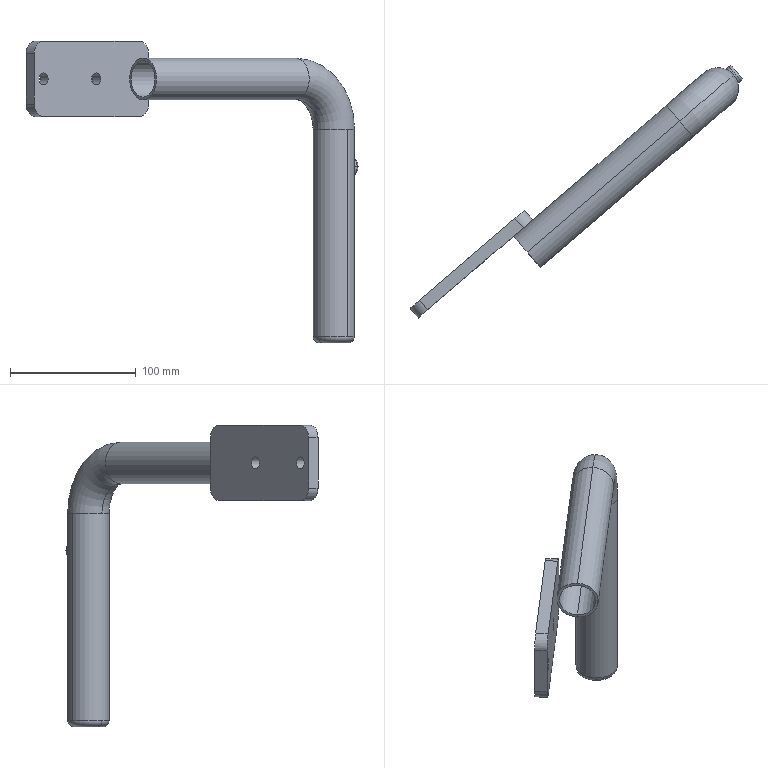Component | SolidWorks | Handle-1 | 2 solids | 39 faces | volume 155457 mm3 | cylinder 20 | plane 11 | torus 8 | commonest cylinder face diameters 15 x4 29 x4 33 x4 9.5 x4 20 x4 | material Stainless Steel